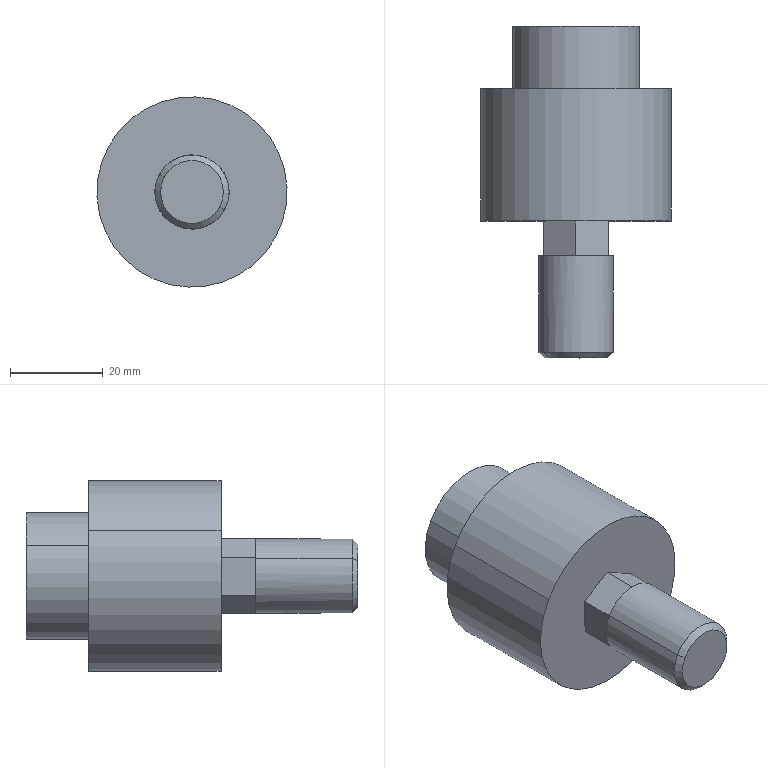Component | SolidWorks | FloatingJointSMCJA50-16-150-1 | 1 solid | 35 faces | box 41 x 71.5 x 41 mm | volume 48926 mm3 | plane 23 | cylinder 8 | cone 4 | commonest cylinder face diameters 41 x2 27.333 x2 16 x2 13.84 x2
STEP:
#1=CARTESIAN_POINT('',(0.08017,-1.417,7.279));
#2=VERTEX_POINT('',#1);
#3=CARTESIAN_POINT('',(1.495,-1.417,6.501));
#4=VERTEX_POINT('',#3);
#5=CARTESIAN_POINT('',(0.7874,-1.417,6.89));
#6=DIRECTION('',(-0.,1.,-0.));
#7=DIRECTION('',(-0.8763,0.,0.4818));
#8=AXIS2_PLACEMENT_3D('',#5,#6,#7);
#9=CIRCLE('',#8,0.8071);
#10=EDGE_CURVE('',#2,#4,#9,.T.);
#11=ORIENTED_EDGE('',*,*,#10,.T.);
#12=CARTESIAN_POINT('',(1.495,-0.2953,6.501));
#13=VERTEX_POINT('',#12);
#14=CARTESIAN_POINT('',(1.495,-0.8563,6.501));
#15=DIRECTION('',(-0.,1.,-0.));
#16=VECTOR('',#15,39.37);
#17=LINE('',#14,#16);
#18=EDGE_CURVE('',#4,#13,#17,.T.);
#19=ORIENTED_EDGE('',*,*,#18,.T.);
#20=CARTESIAN_POINT('',(0.08017,-0.2953,7.279));
#21=VERTEX_POINT('',#20);
#22=CARTESIAN_POINT('',(0.7874,-0.2953,6.89));
#23=DIRECTION('',(0.,-1.,0.));
#24=DIRECTION('',(-0.8763,0.,0.4818));
#25=AXIS2_PLACEMENT_3D('',#22,#23,#24);
#26=CIRCLE('',#25,0.8071);
#27=EDGE_CURVE('',#13,#21,#26,.T.);
#28=ORIENTED_EDGE('',*,*,#27,.T.);
#29=CARTESIAN_POINT('',(0.08017,-0.8563,7.279));
#30=DIRECTION('',(-0.,1.,-0.));
#31=VECTOR('',#30,39.37);
#32=LINE('',#29,#31);
#33=EDGE_CURVE('',#2,#21,#32,.T.);
#34=ORIENTED_EDGE('',*,*,#33,.F.);
#35=EDGE_LOOP('',(#11,#19,#28,#34));
#36=FACE_OUTER_BOUND('',#35,.T.);
#37=CARTESIAN_POINT('',(0.7874,-0.8563,6.89));
#38=DIRECTION('',(-0.,1.,-0.));
#39=DIRECTION('',(-0.8763,0.,0.4818));
#40=AXIS2_PLACEMENT_3D('',#37,#38,#39);
#41=CYLINDRICAL_SURFACE('',#40,0.8071);
#42=ADVANCED_FACE('',(#36),#41,.T.);
#43=CARTESIAN_POINT('',(1.259,-0.2953,6.631));
#44=VERTEX_POINT('',#43);
#45=CARTESIAN_POINT('',(0.3159,-0.2953,7.149));
#46=VERTEX_POINT('',#45);
#47=CARTESIAN_POINT('',(0.7874,-0.2953,6.89));
#48=DIRECTION('',(0.,-1.,0.));
#49=DIRECTION('',(-0.8763,0.,0.4818));
#50=AXIS2_PLACEMENT_3D('',#47,#48,#49);
#51=CIRCLE('',#50,0.5381);
#52=EDGE_CURVE('',#44,#46,#51,.T.);
#53=ORIENTED_EDGE('',*,*,#52,.F.);
#54=CARTESIAN_POINT('',(1.259,0.2362,6.631));
#55=VERTEX_POINT('',#54);
#56=CARTESIAN_POINT('',(1.259,-0.02953,6.631));
#57=DIRECTION('',(-0.,1.,-0.));
#58=VECTOR('',#57,39.37);
#59=LINE('',#56,#58);
#60=EDGE_CURVE('',#44,#55,#59,.T.);
#61=ORIENTED_EDGE('',*,*,#60,.T.);
#62=CARTESIAN_POINT('',(0.3159,0.2362,7.149));
#63=VERTEX_POINT('',#62);
#64=CARTESIAN_POINT('',(0.7874,0.2362,6.89));
#65=DIRECTION('',(0.,-1.,0.));
#66=DIRECTION('',(-0.8763,0.,0.4818));
#67=AXIS2_PLACEMENT_3D('',#64,#65,#66);
#68=CIRCLE('',#67,0.5381);
#69=EDGE_CURVE('',#55,#63,#68,.T.);
#70=ORIENTED_EDGE('',*,*,#69,.T.);
#71=CARTESIAN_POINT('',(0.3159,-0.02953,7.149));
#72=DIRECTION('',(-0.,1.,-0.));
#73=VECTOR('',#72,39.37);
#74=LINE('',#71,#73);
#75=EDGE_CURVE('',#46,#63,#74,.T.);
#76=ORIENTED_EDGE('',*,*,#75,.F.);
#77=EDGE_LOOP('',(#53,#61,#70,#76));
#78=FACE_OUTER_BOUND('',#77,.T.);
#79=CARTESIAN_POINT('',(0.7874,-0.02953,6.89));
#80=DIRECTION('',(-0.,1.,-0.));
#81=DIRECTION('',(-0.8763,0.,0.4818));
#82=AXIS2_PLACEMENT_3D('',#79,#80,#81);
#83=CYLINDRICAL_SURFACE('',#82,0.5381);
#84=ADVANCED_FACE('',(#78),#83,.T.);
#85=CARTESIAN_POINT('',(0.5114,-2.531,7.042));
#86=VERTEX_POINT('',#85);
#87=CARTESIAN_POINT('',(1.063,-2.531,6.738));
#88=VERTEX_POINT('',#87);
#89=CARTESIAN_POINT('',(0.7874,-2.531,6.89));
#90=DIRECTION('',(-0.,1.,-0.));
#91=DIRECTION('',(-0.8763,0.,0.4818));
#92=AXIS2_PLACEMENT_3D('',#89,#90,#91);
#93=CIRCLE('',#92,0.315);
#94=EDGE_CURVE('',#86,#88,#93,.T.);
#95=ORIENTED_EDGE('',*,*,#94,.T.);
#96=CARTESIAN_POINT('',(1.063,-1.713,6.738));
#97=VERTEX_POINT('',#96);
#98=CARTESIAN_POINT('',(1.063,-2.122,6.738));
#99=DIRECTION('',(-0.,1.,-0.));
#100=VECTOR('',#99,39.37);
#101=LINE('',#98,#100);
#102=EDGE_CURVE('',#88,#97,#101,.T.);
#103=ORIENTED_EDGE('',*,*,#102,.T.);
#104=CARTESIAN_POINT('',(1.066,-1.713,6.743));
#105=VERTEX_POINT('',#104);
#106=CARTESIAN_POINT('',(0.7874,-1.713,6.89));
#107=DIRECTION('',(-0.,1.,-0.));
#108=DIRECTION('',(-0.8763,0.,0.4818));
#109=AXIS2_PLACEMENT_3D('',#106,#107,#108);
#110=CIRCLE('',#109,0.315);
#111=EDGE_CURVE('',#105,#97,#110,.T.);
#112=ORIENTED_EDGE('',*,*,#111,.F.);
#113=CARTESIAN_POINT('',(1.06,-1.713,7.048));
#114=VERTEX_POINT('',#113);
#115=CARTESIAN_POINT('',(0.7874,-1.713,6.89));
#116=DIRECTION('',(-0.,1.,-0.));
#117=DIRECTION('',(-0.8763,0.,0.4818));
#118=AXIS2_PLACEMENT_3D('',#115,#116,#117);
#119=CIRCLE('',#118,0.315);
#120=EDGE_CURVE('',#114,#105,#119,.T.);
#121=ORIENTED_EDGE('',*,*,#120,.F.);
#122=CARTESIAN_POINT('',(1.054,-1.713,7.058));
#123=VERTEX_POINT('',#122);
#124=CARTESIAN_POINT('',(0.7874,-1.713,6.89));
#125=DIRECTION('',(-0.,1.,-0.));
#126=DIRECTION('',(-0.8763,0.,0.4818));
#127=AXIS2_PLACEMENT_3D('',#124,#125,#126);
#128=CIRCLE('',#127,0.315);
#129=EDGE_CURVE('',#123,#114,#128,.T.);
#130=ORIENTED_EDGE('',*,*,#129,.F.);
#131=CARTESIAN_POINT('',(0.7866,-1.713,7.205));
#132=VERTEX_POINT('',#131);
#133=CARTESIAN_POINT('',(0.7874,-1.713,6.89));
#134=DIRECTION('',(-0.,1.,-0.));
#135=DIRECTION('',(-0.8763,0.,0.4818));
#136=AXIS2_PLACEMENT_3D('',#133,#134,#135);
#137=CIRCLE('',#136,0.315);
#138=EDGE_CURVE('',#132,#123,#137,.T.);
#139=ORIENTED_EDGE('',*,*,#138,.F.);
#140=CARTESIAN_POINT('',(0.7751,-1.713,7.204));
#141=VERTEX_POINT('',#140);
#142=CARTESIAN_POINT('',(0.7874,-1.713,6.89));
#143=DIRECTION('',(-0.,1.,-0.));
#144=DIRECTION('',(-0.8763,0.,0.4818));
#145=AXIS2_PLACEMENT_3D('',#142,#143,#144);
#146=CIRCLE('',#145,0.315);
#147=EDGE_CURVE('',#141,#132,#146,.T.);
#148=ORIENTED_EDGE('',*,*,#147,.F.);
#149=CARTESIAN_POINT('',(0.5142,-1.713,7.047));
#150=VERTEX_POINT('',#149);
#151=CARTESIAN_POINT('',(0.7874,-1.713,6.89));
#152=DIRECTION('',(-0.,1.,-0.));
#153=DIRECTION('',(-0.8763,0.,0.4818));
#154=AXIS2_PLACEMENT_3D('',#151,#152,#153);
#155=CIRCLE('',#154,0.315);
#156=EDGE_CURVE('',#150,#141,#155,.T.);
#157=ORIENTED_EDGE('',*,*,#156,.F.);
#158=CARTESIAN_POINT('',(0.5114,-1.713,7.042));
#159=VERTEX_POINT('',#158);
#160=CARTESIAN_POINT('',(0.7874,-1.713,6.89));
#161=DIRECTION('',(-0.,1.,-0.));
#162=DIRECTION('',(-0.8763,0.,0.4818));
#163=AXIS2_PLACEMENT_3D('',#160,#161,#162);
#164=CIRCLE('',#163,0.315);
#165=EDGE_CURVE('',#159,#150,#164,.T.);
#166=ORIENTED_EDGE('',*,*,#165,.F.);
#167=CARTESIAN_POINT('',(0.5114,-2.122,7.042));
#168=DIRECTION('',(-0.,1.,-0.));
#169=VECTOR('',#168,39.37);
#170=LINE('',#167,#169);
#171=EDGE_CURVE('',#86,#159,#170,.T.);
#172=ORIENTED_EDGE('',*,*,#171,.F.);
#173=EDGE_LOOP('',(#95,#103,#112,#121,#130,#139,#148,#157,#166,#172));
#174=FACE_OUTER_BOUND('',#173,.T.);
#175=CARTESIAN_POINT('',(0.7874,-2.122,6.89));
#176=DIRECTION('',(-0.,1.,-0.));
#177=DIRECTION('',(-0.8763,0.,0.4818));
#178=AXIS2_PLACEMENT_3D('',#175,#176,#177);
#179=CYLINDRICAL_SURFACE('',#178,0.315);
#180=ADVANCED_FACE('',(#174),#179,.T.);
#181=CARTESIAN_POINT('',(1.026,0.1937,6.758));
#182=VERTEX_POINT('',#181);
#183=CARTESIAN_POINT('',(0.5487,0.1937,7.021));
#184=VERTEX_POINT('',#183);
#185=CARTESIAN_POINT('',(0.7874,0.1937,6.89));
#186=DIRECTION('',(-0.,1.,-0.));
#187=DIRECTION('',(0.4818,0.,0.8763));
#188=AXIS2_PLACEMENT_3D('',#185,#186,#187);
#189=CIRCLE('',#188,0.2724);
#190=EDGE_CURVE('',#182,#184,#189,.T.);
#191=ORIENTED_EDGE('',*,*,#190,.F.);
#192=CARTESIAN_POINT('',(1.063,0.2362,6.738));
#193=VERTEX_POINT('',#192);
#194=CARTESIAN_POINT('',(1.063,0.2362,6.738));
#195=DIRECTION('',(0.6196,0.7071,-0.3407));
#196=VECTOR('',#195,39.37);
#197=LINE('',#194,#196);
#198=EDGE_CURVE('',#182,#193,#197,.T.);
#199=ORIENTED_EDGE('',*,*,#198,.T.);
#200=CARTESIAN_POINT('',(0.5114,0.2362,7.042));
#201=VERTEX_POINT('',#200);
#202=CARTESIAN_POINT('',(0.7874,0.2362,6.89));
#203=DIRECTION('',(0.,-1.,0.));
#204=DIRECTION('',(-0.8763,0.,0.4818));
#205=AXIS2_PLACEMENT_3D('',#202,#203,#204);
#206=CIRCLE('',#205,0.315);
#207=EDGE_CURVE('',#201,#193,#206,.T.);
#208=ORIENTED_EDGE('',*,*,#207,.F.);
#209=CARTESIAN_POINT('',(0.5114,0.2362,7.042));
#210=DIRECTION('',(-0.6196,0.7071,0.3407));
#211=VECTOR('',#210,39.37);
#212=LINE('',#209,#211);
#213=EDGE_CURVE('',#184,#201,#212,.T.);
#214=ORIENTED_EDGE('',*,*,#213,.F.);
#215=EDGE_LOOP('',(#191,#199,#208,#214));
#216=FACE_OUTER_BOUND('',#215,.T.);
#217=CARTESIAN_POINT('',(0.7874,0.2362,6.89));
#218=DIRECTION('',(-0.,1.,-0.));
#219=DIRECTION('',(-0.8763,0.,0.4818));
#220=AXIS2_PLACEMENT_3D('',#217,#218,#219);
#221=CONICAL_SURFACE('',#220,0.315,0.7854);
#222=ADVANCED_FACE('',(#216),#221,.F.);
#223=CARTESIAN_POINT('',(0.5537,-2.579,7.018));
#224=VERTEX_POINT('',#223);
#225=CARTESIAN_POINT('',(1.021,-2.579,6.761));
#226=VERTEX_POINT('',#225);
#227=CARTESIAN_POINT('',(0.7874,-2.579,6.89));
#228=DIRECTION('',(-0.,1.,-0.));
#229=DIRECTION('',(-0.8763,0.,0.4818));
#230=AXIS2_PLACEMENT_3D('',#227,#228,#229);
#231=CIRCLE('',#230,0.2667);
#232=EDGE_CURVE('',#224,#226,#231,.T.);
#233=ORIENTED_EDGE('',*,*,#232,.T.);
#234=CARTESIAN_POINT('',(1.063,-2.531,6.738));
#235=DIRECTION('',(0.6196,0.7071,-0.3407));
#236=VECTOR('',#235,39.37);
#237=LINE('',#234,#236);
#238=EDGE_CURVE('',#226,#88,#237,.T.);
#239=ORIENTED_EDGE('',*,*,#238,.T.);
#240=ORIENTED_EDGE('',*,*,#94,.F.);
#241=CARTESIAN_POINT('',(0.5114,-2.531,7.042));
#242=DIRECTION('',(-0.6196,0.7071,0.3407));
#243=VECTOR('',#242,39.37);
#244=LINE('',#241,#243);
#245=EDGE_CURVE('',#224,#86,#244,.T.);
#246=ORIENTED_EDGE('',*,*,#245,.F.);
#247=EDGE_LOOP('',(#233,#239,#240,#246));
#248=FACE_OUTER_BOUND('',#247,.T.);
#249=CARTESIAN_POINT('',(0.7874,-2.531,6.89));
#250=DIRECTION('',(-0.,1.,-0.));
#251=DIRECTION('',(-0.8763,0.,0.4818));
#252=AXIS2_PLACEMENT_3D('',#249,#250,#251);
#253=CONICAL_SURFACE('',#252,0.315,0.7854);
#254=ADVANCED_FACE('',(#248),#253,.T.);
#255=CARTESIAN_POINT('',(1.026,-0.3543,6.758));
#256=VERTEX_POINT('',#255);
#257=CARTESIAN_POINT('',(0.5487,-0.3543,7.021));
#258=VERTEX_POINT('',#257);
#259=CARTESIAN_POINT('',(0.7874,-0.3543,6.89));
#260=DIRECTION('',(-0.,1.,-0.));
#261=DIRECTION('',(-0.8763,0.,0.4818));
#262=AXIS2_PLACEMENT_3D('',#259,#260,#261);
#263=CIRCLE('',#262,0.2724);
#264=EDGE_CURVE('',#256,#258,#263,.T.);
#265=ORIENTED_EDGE('',*,*,#264,.F.);
#266=CARTESIAN_POINT('',(1.026,-0.08031,6.758));
#267=DIRECTION('',(-0.,1.,-0.));
#268=VECTOR('',#267,39.37);
#269=LINE('',#266,#268);
#270=EDGE_CURVE('',#256,#182,#269,.T.);
#271=ORIENTED_EDGE('',*,*,#270,.T.);
#272=ORIENTED_EDGE('',*,*,#190,.T.);
#273=CARTESIAN_POINT('',(0.5487,-0.08031,7.021));
#274=DIRECTION('',(-0.,1.,-0.));
#275=VECTOR('',#274,39.37);
#276=LINE('',#273,#275);
#277=EDGE_CURVE('',#258,#184,#276,.T.);
#278=ORIENTED_EDGE('',*,*,#277,.F.);
#279=EDGE_LOOP('',(#265,#271,#272,#278));
#280=FACE_OUTER_BOUND('',#279,.T.);
#281=CARTESIAN_POINT('',(0.7874,-0.08031,6.89));
#282=DIRECTION('',(-0.,1.,-0.));
#283=DIRECTION('',(-0.8763,0.,0.4818));
#284=AXIS2_PLACEMENT_3D('',#281,#282,#283);
#285=CYLINDRICAL_SURFACE('',#284,0.2724);
#286=ADVANCED_FACE('',(#280),#285,.F.);
#287=ORIENTED_EDGE('',*,*,#18,.F.);
#288=CARTESIAN_POINT('',(0.7874,-1.417,6.89));
#289=DIRECTION('',(-0.,1.,-0.));
#290=DIRECTION('',(-0.8763,0.,0.4818));
#291=AXIS2_PLACEMENT_3D('',#288,#289,#290);
#292=CIRCLE('',#291,0.8071);
#293=EDGE_CURVE('',#4,#2,#292,.T.);
#294=ORIENTED_EDGE('',*,*,#293,.T.);
#295=ORIENTED_EDGE('',*,*,#33,.T.);
#296=CARTESIAN_POINT('',(0.7874,-0.2953,6.89));
#297=DIRECTION('',(0.,-1.,0.));
#298=DIRECTION('',(-0.8763,0.,0.4818));
#299=AXIS2_PLACEMENT_3D('',#296,#297,#298);
#300=CIRCLE('',#299,0.8071);
#301=EDGE_CURVE('',#21,#13,#300,.T.);
#302=ORIENTED_EDGE('',*,*,#301,.T.);
#303=EDGE_LOOP('',(#287,#294,#295,#302));
#304=FACE_OUTER_BOUND('',#303,.T.);
#305=CARTESIAN_POINT('',(0.7874,-0.8563,6.89));
#306=DIRECTION('',(-0.,1.,-0.));
#307=DIRECTION('',(-0.8763,0.,0.4818));
#308=AXIS2_PLACEMENT_3D('',#305,#306,#307);
#309=CYLINDRICAL_SURFACE('',#308,0.8071);
#310=ADVANCED_FACE('',(#304),#309,.T.);
#311=ORIENTED_EDGE('',*,*,#10,.F.);
#312=ORIENTED_EDGE('',*,*,#293,.F.);
#313=EDGE_LOOP('',(#311,#312));
#314=FACE_OUTER_BOUND('',#313,.T.);
#315=CARTESIAN_POINT('',(1.066,-1.417,6.736));
#316=VERTEX_POINT('',#315);
#317=CARTESIAN_POINT('',(0.794,-1.417,6.572));
#318=VERTEX_POINT('',#317);
#319=CARTESIAN_POINT('',(1.066,-1.417,6.736));
#320=DIRECTION('',(-0.8554,-0.,-0.518));
#321=VECTOR('',#320,39.37);
#322=LINE('',#319,#321);
#323=EDGE_CURVE('',#316,#318,#322,.T.);
#324=ORIENTED_EDGE('',*,*,#323,.T.);
#325=CARTESIAN_POINT('',(0.5152,-1.417,6.725));
#326=VERTEX_POINT('',#325);
#327=CARTESIAN_POINT('',(0.6546,-1.417,6.648));
#328=DIRECTION('',(-0.8763,0.,0.4818));
#329=VECTOR('',#328,39.37);
#330=LINE('',#327,#329);
#331=EDGE_CURVE('',#318,#326,#330,.T.);
#332=ORIENTED_EDGE('',*,*,#331,.T.);
#333=CARTESIAN_POINT('',(0.5086,-1.417,7.043));
#334=VERTEX_POINT('',#333);
#335=CARTESIAN_POINT('',(0.5152,-1.417,6.725));
#336=DIRECTION('',(-0.02087,0.,0.9998));
#337=VECTOR('',#336,39.37);
#338=LINE('',#335,#337);
#339=EDGE_CURVE('',#326,#334,#338,.T.);
#340=ORIENTED_EDGE('',*,*,#339,.T.);
#341=CARTESIAN_POINT('',(0.7808,-1.417,7.208));
#342=VERTEX_POINT('',#341);
#343=CARTESIAN_POINT('',(0.5086,-1.417,7.043));
#344=DIRECTION('',(0.8554,0.,0.518));
#345=VECTOR('',#344,39.37);
#346=LINE('',#343,#345);
#347=EDGE_CURVE('',#334,#342,#346,.T.);
#348=ORIENTED_EDGE('',*,*,#347,.T.);
#349=CARTESIAN_POINT('',(1.06,-1.417,7.055));
#350=VERTEX_POINT('',#349);
#351=CARTESIAN_POINT('',(0.9202,-1.417,7.131));
#352=DIRECTION('',(0.8763,-0.,-0.4818));
#353=VECTOR('',#352,39.37);
#354=LINE('',#351,#353);
#355=EDGE_CURVE('',#342,#350,#354,.T.);
#356=ORIENTED_EDGE('',*,*,#355,.T.);
#357=CARTESIAN_POINT('',(1.06,-1.417,7.055));
#358=DIRECTION('',(0.02087,-0.,-0.9998));
#359=VECTOR('',#358,39.37);
#360=LINE('',#357,#359);
#361=EDGE_CURVE('',#350,#316,#360,.T.);
#362=ORIENTED_EDGE('',*,*,#361,.T.);
#363=EDGE_LOOP('',(#324,#332,#340,#348,#356,#362));
#364=FACE_BOUND('',#363,.T.);
#365=CARTESIAN_POINT('',(0.9818,-1.417,7.243));
#366=DIRECTION('',(0.,-1.,0.));
#367=DIRECTION('',(0.8763,-0.,-0.4818));
#368=AXIS2_PLACEMENT_3D('',#365,#366,#367);
#369=PLANE('',#368);
#370=ADVANCED_FACE('',(#314,#364),#369,.T.);
#371=CARTESIAN_POINT('',(0.7874,-0.2953,6.89));
#372=DIRECTION('',(0.,-1.,0.));
#373=DIRECTION('',(-0.8763,0.,0.4818));
#374=AXIS2_PLACEMENT_3D('',#371,#372,#373);
#375=CIRCLE('',#374,0.5381);
#376=EDGE_CURVE('',#46,#44,#375,.T.);
#377=ORIENTED_EDGE('',*,*,#376,.T.);
#378=ORIENTED_EDGE('',*,*,#52,.T.);
#379=EDGE_LOOP('',(#377,#378));
#380=FACE_BOUND('',#379,.T.);
#381=ORIENTED_EDGE('',*,*,#301,.F.);
#382=ORIENTED_EDGE('',*,*,#27,.F.);
#383=EDGE_LOOP('',(#381,#382));
#384=FACE_OUTER_BOUND('',#383,.T.);
#385=CARTESIAN_POINT('',(1.111,-0.2953,7.479));
#386=DIRECTION('',(-0.,1.,-0.));
#387=DIRECTION('',(-0.8763,0.,0.4818));
#388=AXIS2_PLACEMENT_3D('',#385,#386,#387);
#389=PLANE('',#388);
#390=ADVANCED_FACE('',(#380,#384),#389,.T.);
#391=ORIENTED_EDGE('',*,*,#331,.F.);
#392=CARTESIAN_POINT('',(0.794,-1.713,6.572));
#393=VERTEX_POINT('',#392);
#394=CARTESIAN_POINT('',(0.794,-1.417,6.572));
#395=DIRECTION('',(0.,-1.,0.));
#396=VECTOR('',#395,39.37);
#397=LINE('',#394,#396);
#398=EDGE_CURVE('',#318,#393,#397,.T.);
#399=ORIENTED_EDGE('',*,*,#398,.T.);
#400=CARTESIAN_POINT('',(0.7882,-1.713,6.575));
#401=VERTEX_POINT('',#400);
#402=CARTESIAN_POINT('',(0.794,-1.713,6.572));
#403=DIRECTION('',(-0.8763,0.,0.4818));
#404=VECTOR('',#403,39.37);
#405=LINE('',#402,#404);
#406=EDGE_CURVE('',#393,#401,#405,.T.);
#407=ORIENTED_EDGE('',*,*,#406,.T.);
#408=CARTESIAN_POINT('',(0.521,-1.713,6.722));
#409=VERTEX_POINT('',#408);
#410=CARTESIAN_POINT('',(0.794,-1.713,6.572));
#411=DIRECTION('',(-0.8763,0.,0.4818));
#412=VECTOR('',#411,39.37);
#413=LINE('',#410,#412);
#414=EDGE_CURVE('',#401,#409,#413,.T.);
#415=ORIENTED_EDGE('',*,*,#414,.T.);
#416=CARTESIAN_POINT('',(0.5152,-1.713,6.725));
#417=VERTEX_POINT('',#416);
#418=CARTESIAN_POINT('',(0.794,-1.713,6.572));
#419=DIRECTION('',(-0.8763,0.,0.4818));
#420=VECTOR('',#419,39.37);
#421=LINE('',#418,#420);
#422=EDGE_CURVE('',#409,#417,#421,.T.);
#423=ORIENTED_EDGE('',*,*,#422,.T.);
#424=CARTESIAN_POINT('',(0.5152,-1.417,6.725));
#425=DIRECTION('',(-0.,1.,-0.));
#426=VECTOR('',#425,39.37);
#427=LINE('',#424,#426);
#428=EDGE_CURVE('',#417,#326,#427,.T.);
#429=ORIENTED_EDGE('',*,*,#428,.T.);
#430=EDGE_LOOP('',(#391,#399,#407,#415,#423,#429));
#431=FACE_OUTER_BOUND('',#430,.T.);
#432=CARTESIAN_POINT('',(0.794,-1.417,6.572));
#433=DIRECTION('',(-0.4818,-0.,-0.8763));
#434=DIRECTION('',(-0.,1.,-0.));
#435=AXIS2_PLACEMENT_3D('',#432,#433,#434);
#436=PLANE('',#435);
#437=ADVANCED_FACE('',(#431),#436,.T.);
#438=ORIENTED_EDGE('',*,*,#323,.F.);
#439=CARTESIAN_POINT('',(1.066,-1.713,6.736));
#440=VERTEX_POINT('',#439);
#441=CARTESIAN_POINT('',(1.066,-1.417,6.736));
#442=DIRECTION('',(0.,-1.,0.));
#443=VECTOR('',#442,39.37);
#444=LINE('',#441,#443);
#445=EDGE_CURVE('',#316,#440,#444,.T.);
#446=ORIENTED_EDGE('',*,*,#445,.T.);
#447=CARTESIAN_POINT('',(1.061,-1.713,6.733));
#448=VERTEX_POINT('',#447);
#449=CARTESIAN_POINT('',(1.066,-1.713,6.736));
#450=DIRECTION('',(-0.8554,-0.,-0.518));
#451=VECTOR('',#450,39.37);
#452=LINE('',#449,#451);
#453=EDGE_CURVE('',#440,#448,#452,.T.);
#454=ORIENTED_EDGE('',*,*,#453,.T.);
#455=CARTESIAN_POINT('',(0.7997,-1.713,6.575));
#456=VERTEX_POINT('',#455);
#457=CARTESIAN_POINT('',(1.066,-1.713,6.736));
#458=DIRECTION('',(-0.8554,-0.,-0.518));
#459=VECTOR('',#458,39.37);
#460=LINE('',#457,#459);
#461=EDGE_CURVE('',#448,#456,#460,.T.);
#462=ORIENTED_EDGE('',*,*,#461,.T.);
#463=CARTESIAN_POINT('',(1.066,-1.713,6.736));
#464=DIRECTION('',(-0.8554,-0.,-0.518));
#465=VECTOR('',#464,39.37);
#466=LINE('',#463,#465);
#467=EDGE_CURVE('',#456,#393,#466,.T.);
#468=ORIENTED_EDGE('',*,*,#467,.T.);
#469=ORIENTED_EDGE('',*,*,#398,.F.);
#470=EDGE_LOOP('',(#438,#446,#454,#462,#468,#469));
#471=FACE_OUTER_BOUND('',#470,.T.);
#472=CARTESIAN_POINT('',(1.066,-1.417,6.736));
#473=DIRECTION('',(0.518,-0.,-0.8554));
#474=DIRECTION('',(0.8554,0.,0.518));
#475=AXIS2_PLACEMENT_3D('',#472,#473,#474);
#476=PLANE('',#475);
#477=ADVANCED_FACE('',(#471),#476,.T.);
#478=ORIENTED_EDGE('',*,*,#361,.F.);
#479=CARTESIAN_POINT('',(1.06,-1.713,7.055));
#480=VERTEX_POINT('',#479);
#481=CARTESIAN_POINT('',(1.06,-1.417,7.055));
#482=DIRECTION('',(0.,-1.,0.));
#483=VECTOR('',#482,39.37);
#484=LINE('',#481,#483);
#485=EDGE_CURVE('',#350,#480,#484,.T.);
#486=ORIENTED_EDGE('',*,*,#485,.T.);
#487=CARTESIAN_POINT('',(1.06,-1.713,7.055));
#488=DIRECTION('',(0.02087,-0.,-0.9998));
#489=VECTOR('',#488,39.37);
#490=LINE('',#487,#489);
#491=EDGE_CURVE('',#480,#114,#490,.T.);
#492=ORIENTED_EDGE('',*,*,#491,.T.);
#493=CARTESIAN_POINT('',(1.06,-1.713,7.055));
#494=DIRECTION('',(0.02087,-0.,-0.9998));
#495=VECTOR('',#494,39.37);
#496=LINE('',#493,#495);
#497=EDGE_CURVE('',#114,#105,#496,.T.);
#498=ORIENTED_EDGE('',*,*,#497,.T.);
#499=CARTESIAN_POINT('',(1.06,-1.713,7.055));
#500=DIRECTION('',(0.02087,-0.,-0.9998));
#501=VECTOR('',#500,39.37);
#502=LINE('',#499,#501);
#503=EDGE_CURVE('',#105,#440,#502,.T.);
#504=ORIENTED_EDGE('',*,*,#503,.T.);
#505=ORIENTED_EDGE('',*,*,#445,.F.);
#506=EDGE_LOOP('',(#478,#486,#492,#498,#504,#505));
#507=FACE_OUTER_BOUND('',#506,.T.);
#508=CARTESIAN_POINT('',(1.06,-1.417,7.055));
#509=DIRECTION('',(0.9998,0.,0.02087));
#510=DIRECTION('',(-0.02087,0.,0.9998));
#511=AXIS2_PLACEMENT_3D('',#508,#509,#510);
#512=PLANE('',#511);
#513=ADVANCED_FACE('',(#507),#512,.T.);
#514=ORIENTED_EDGE('',*,*,#355,.F.);
#515=CARTESIAN_POINT('',(0.7808,-1.713,7.208));
#516=VERTEX_POINT('',#515);
#517=CARTESIAN_POINT('',(0.7808,-1.417,7.208));
#518=DIRECTION('',(0.,-1.,0.));
#519=VECTOR('',#518,39.37);
#520=LINE('',#517,#519);
#521=EDGE_CURVE('',#342,#516,#520,.T.);
#522=ORIENTED_EDGE('',*,*,#521,.T.);
#523=CARTESIAN_POINT('',(0.7808,-1.713,7.208));
#524=DIRECTION('',(0.8763,-0.,-0.4818));
#525=VECTOR('',#524,39.37);
#526=LINE('',#523,#525);
#527=EDGE_CURVE('',#516,#132,#526,.T.);
#528=ORIENTED_EDGE('',*,*,#527,.T.);
#529=CARTESIAN_POINT('',(0.7808,-1.713,7.208));
#530=DIRECTION('',(0.8763,-0.,-0.4818));
#531=VECTOR('',#530,39.37);
#532=LINE('',#529,#531);
#533=EDGE_CURVE('',#132,#123,#532,.T.);
#534=ORIENTED_EDGE('',*,*,#533,.T.);
#535=CARTESIAN_POINT('',(0.7808,-1.713,7.208));
#536=DIRECTION('',(0.8763,-0.,-0.4818));
#537=VECTOR('',#536,39.37);
#538=LINE('',#535,#537);
#539=EDGE_CURVE('',#123,#480,#538,.T.);
#540=ORIENTED_EDGE('',*,*,#539,.T.);
#541=ORIENTED_EDGE('',*,*,#485,.F.);
#542=EDGE_LOOP('',(#514,#522,#528,#534,#540,#541));
#543=FACE_OUTER_BOUND('',#542,.T.);
#544=CARTESIAN_POINT('',(0.7808,-1.417,7.208));
#545=DIRECTION('',(0.4818,0.,0.8763));
#546=DIRECTION('',(0.,-1.,0.));
#547=AXIS2_PLACEMENT_3D('',#544,#545,#546);
#548=PLANE('',#547);
#549=ADVANCED_FACE('',(#543),#548,.T.);
#550=ORIENTED_EDGE('',*,*,#347,.F.);
#551=CARTESIAN_POINT('',(0.5086,-1.713,7.043));
#552=VERTEX_POINT('',#551);
#553=CARTESIAN_POINT('',(0.5086,-1.417,7.043));
#554=DIRECTION('',(0.,-1.,0.));
#555=VECTOR('',#554,39.37);
#556=LINE('',#553,#555);
#557=EDGE_CURVE('',#334,#552,#556,.T.);
#558=ORIENTED_EDGE('',*,*,#557,.T.);
#559=CARTESIAN_POINT('',(0.5086,-1.713,7.043));
#560=DIRECTION('',(0.8554,0.,0.518));
#561=VECTOR('',#560,39.37);
#562=LINE('',#559,#561);
#563=EDGE_CURVE('',#552,#150,#562,.T.);
#564=ORIENTED_EDGE('',*,*,#563,.T.);
#565=CARTESIAN_POINT('',(0.5086,-1.713,7.043));
#566=DIRECTION('',(0.8554,0.,0.518));
#567=VECTOR('',#566,39.37);
#568=LINE('',#565,#567);
#569=EDGE_CURVE('',#150,#141,#568,.T.);
#570=ORIENTED_EDGE('',*,*,#569,.T.);
#571=CARTESIAN_POINT('',(0.5086,-1.713,7.043));
#572=DIRECTION('',(0.8554,0.,0.518));
#573=VECTOR('',#572,39.37);
#574=LINE('',#571,#573);
#575=EDGE_CURVE('',#141,#516,#574,.T.);
#576=ORIENTED_EDGE('',*,*,#575,.T.);
#577=ORIENTED_EDGE('',*,*,#521,.F.);
#578=EDGE_LOOP('',(#550,#558,#564,#570,#576,#577));
#579=FACE_OUTER_BOUND('',#578,.T.);
#580=CARTESIAN_POINT('',(0.5086,-1.417,7.043));
#581=DIRECTION('',(-0.518,0.,0.8554));
#582=DIRECTION('',(-0.8554,-0.,-0.518));
#583=AXIS2_PLACEMENT_3D('',#580,#581,#582);
#584=PLANE('',#583);
#585=ADVANCED_FACE('',(#579),#584,.T.);
#586=ORIENTED_EDGE('',*,*,#339,.F.);
#587=ORIENTED_EDGE('',*,*,#428,.F.);
#588=CARTESIAN_POINT('',(0.5151,-1.713,6.732));
#589=VERTEX_POINT('',#588);
#590=CARTESIAN_POINT('',(0.5152,-1.713,6.725));
#591=DIRECTION('',(-0.02087,0.,0.9998));
#592=VECTOR('',#591,39.37);
#593=LINE('',#590,#592);
#594=EDGE_CURVE('',#417,#589,#593,.T.);
#595=ORIENTED_EDGE('',*,*,#594,.T.);
#596=CARTESIAN_POINT('',(0.5087,-1.713,7.036));
#597=VERTEX_POINT('',#596);
#598=CARTESIAN_POINT('',(0.5152,-1.713,6.725));
#599=DIRECTION('',(-0.02087,0.,0.9998));
#600=VECTOR('',#599,39.37);
#601=LINE('',#598,#600);
#602=EDGE_CURVE('',#589,#597,#601,.T.);
#603=ORIENTED_EDGE('',*,*,#602,.T.);
#604=CARTESIAN_POINT('',(0.5152,-1.713,6.725));
#605=DIRECTION('',(-0.02087,0.,0.9998));
#606=VECTOR('',#605,39.37);
#607=LINE('',#604,#606);
#608=EDGE_CURVE('',#597,#552,#607,.T.);
#609=ORIENTED_EDGE('',*,*,#608,.T.);
#610=ORIENTED_EDGE('',*,*,#557,.F.);
#611=EDGE_LOOP('',(#586,#587,#595,#603,#609,#610));
#612=FACE_OUTER_BOUND('',#611,.T.);
#613=CARTESIAN_POINT('',(0.5152,-1.417,6.725));
#614=DIRECTION('',(-0.9998,-0.,-0.02087));
#615=DIRECTION('',(0.02087,-0.,-0.9998));
#616=AXIS2_PLACEMENT_3D('',#613,#614,#615);
#617=PLANE('',#616);
#618=ADVANCED_FACE('',(#612),#617,.T.);
#619=ORIENTED_EDGE('',*,*,#60,.F.);
#620=ORIENTED_EDGE('',*,*,#376,.F.);
#621=ORIENTED_EDGE('',*,*,#75,.T.);
#622=CARTESIAN_POINT('',(0.7874,0.2362,6.89));
#623=DIRECTION('',(0.,-1.,0.));
#624=DIRECTION('',(-0.8763,0.,0.4818));
#625=AXIS2_PLACEMENT_3D('',#622,#623,#624);
#626=CIRCLE('',#625,0.5381);
#627=EDGE_CURVE('',#63,#55,#626,.T.);
#628=ORIENTED_EDGE('',*,*,#627,.T.);
#629=EDGE_LOOP('',(#619,#620,#621,#628));
#630=FACE_OUTER_BOUND('',#629,.T.);
#631=CARTESIAN_POINT('',(0.7874,-0.02953,6.89));
#632=DIRECTION('',(-0.,1.,-0.));
#633=DIRECTION('',(-0.8763,0.,0.4818));
#634=AXIS2_PLACEMENT_3D('',#631,#632,#633);
#635=CYLINDRICAL_SURFACE('',#634,0.5381);
#636=ADVANCED_FACE('',(#630),#635,.T.);
#637=ORIENTED_EDGE('',*,*,#594,.F.);
#638=ORIENTED_EDGE('',*,*,#422,.F.);
#639=CARTESIAN_POINT('',(0.7874,-1.713,6.89));
#640=DIRECTION('',(0.,-1.,0.));
#641=DIRECTION('',(-0.8763,0.,0.4818));
#642=AXIS2_PLACEMENT_3D('',#639,#640,#641);
#643=CIRCLE('',#642,0.315);
#644=EDGE_CURVE('',#589,#409,#643,.T.);
#645=ORIENTED_EDGE('',*,*,#644,.F.);
#646=EDGE_LOOP('',(#637,#638,#645));
#647=FACE_OUTER_BOUND('',#646,.T.);
#648=CARTESIAN_POINT('',(0.7874,-1.713,6.89));
#649=DIRECTION('',(0.,-1.,0.));
#650=DIRECTION('',(0.8763,-0.,-0.4818));
#651=AXIS2_PLACEMENT_3D('',#648,#649,#650);
#652=PLANE('',#651);
#653=ADVANCED_FACE('',(#647),#652,.T.);
#654=ORIENTED_EDGE('',*,*,#414,.F.);
#655=CARTESIAN_POINT('',(0.7874,-1.713,6.89));
#656=DIRECTION('',(-0.,1.,-0.));
#657=DIRECTION('',(-0.8763,0.,0.4818));
#658=AXIS2_PLACEMENT_3D('',#655,#656,#657);
#659=CIRCLE('',#658,0.315);
#660=EDGE_CURVE('',#401,#409,#659,.T.);
#661=ORIENTED_EDGE('',*,*,#660,.T.);
#662=EDGE_LOOP('',(#654,#661));
#663=FACE_OUTER_BOUND('',#662,.T.);
#664=CARTESIAN_POINT('',(0.8633,-1.713,7.028));
#665=DIRECTION('',(-0.,1.,-0.));
#666=DIRECTION('',(-0.8763,0.,0.4818));
#667=AXIS2_PLACEMENT_3D('',#664,#665,#666);
#668=PLANE('',#667);
#669=ADVANCED_FACE('',(#663),#668,.T.);
#670=ORIENTED_EDGE('',*,*,#406,.F.);
#671=ORIENTED_EDGE('',*,*,#467,.F.);
#672=CARTESIAN_POINT('',(0.7874,-1.713,6.89));
#673=DIRECTION('',(-0.,1.,-0.));
#674=DIRECTION('',(-0.8763,0.,0.4818));
#675=AXIS2_PLACEMENT_3D('',#672,#673,#674);
#676=CIRCLE('',#675,0.315);
#677=EDGE_CURVE('',#456,#401,#676,.T.);
#678=ORIENTED_EDGE('',*,*,#677,.T.);
#679=EDGE_LOOP('',(#670,#671,#678));
#680=FACE_OUTER_BOUND('',#679,.T.);
#681=CARTESIAN_POINT('',(0.7874,-1.713,6.89));
#682=DIRECTION('',(0.,-1.,0.));
#683=DIRECTION('',(0.8763,-0.,-0.4818));
#684=AXIS2_PLACEMENT_3D('',#681,#682,#683);
#685=PLANE('',#684);
#686=ADVANCED_FACE('',(#680),#685,.T.);
#687=ORIENTED_EDGE('',*,*,#461,.F.);
#688=CARTESIAN_POINT('',(0.7874,-1.713,6.89));
#689=DIRECTION('',(-0.,1.,-0.));
#690=DIRECTION('',(-0.8763,0.,0.4818));
#691=AXIS2_PLACEMENT_3D('',#688,#689,#690);
#692=CIRCLE('',#691,0.315);
#693=EDGE_CURVE('',#448,#456,#692,.T.);
#694=ORIENTED_EDGE('',*,*,#693,.T.);
#695=EDGE_LOOP('',(#687,#694));
#696=FACE_OUTER_BOUND('',#695,.T.);
#697=CARTESIAN_POINT('',(0.8633,-1.713,7.028));
#698=DIRECTION('',(-0.,1.,-0.));
#699=DIRECTION('',(-0.8763,0.,0.4818));
#700=AXIS2_PLACEMENT_3D('',#697,#698,#699);
#701=PLANE('',#700);
#702=ADVANCED_FACE('',(#696),#701,.T.);
#703=ORIENTED_EDGE('',*,*,#453,.F.);
#704=ORIENTED_EDGE('',*,*,#503,.F.);
#705=ORIENTED_EDGE('',*,*,#111,.T.);
#706=CARTESIAN_POINT('',(0.7874,-1.713,6.89));
#707=DIRECTION('',(-0.,1.,-0.));
#708=DIRECTION('',(-0.8763,0.,0.4818));
#709=AXIS2_PLACEMENT_3D('',#706,#707,#708);
#710=CIRCLE('',#709,0.315);
#711=EDGE_CURVE('',#97,#448,#710,.T.);
#712=ORIENTED_EDGE('',*,*,#711,.T.);
#713=EDGE_LOOP('',(#703,#704,#705,#712));
#714=FACE_OUTER_BOUND('',#713,.T.);
#715=CARTESIAN_POINT('',(0.7874,-1.713,6.89));
#716=DIRECTION('',(0.,-1.,0.));
#717=DIRECTION('',(0.8763,-0.,-0.4818));
#718=AXIS2_PLACEMENT_3D('',#715,#716,#717);
#719=PLANE('',#718);
#720=ADVANCED_FACE('',(#714),#719,.T.);
#721=ORIENTED_EDGE('',*,*,#497,.F.);
#722=ORIENTED_EDGE('',*,*,#120,.T.);
#723=EDGE_LOOP('',(#721,#722));
#724=FACE_OUTER_BOUND('',#723,.T.);
#725=CARTESIAN_POINT('',(0.8633,-1.713,7.028));
#726=DIRECTION('',(-0.,1.,-0.));
#727=DIRECTION('',(-0.8763,0.,0.4818));
#728=AXIS2_PLACEMENT_3D('',#725,#726,#727);
#729=PLANE('',#728);
#730=ADVANCED_FACE('',(#724),#729,.T.);
#731=ORIENTED_EDGE('',*,*,#491,.F.);
#732=ORIENTED_EDGE('',*,*,#539,.F.);
#733=ORIENTED_EDGE('',*,*,#129,.T.);
#734=EDGE_LOOP('',(#731,#732,#733));
#735=FACE_OUTER_BOUND('',#734,.T.);
#736=CARTESIAN_POINT('',(0.7874,-1.713,6.89));
#737=DIRECTION('',(0.,-1.,0.));
#738=DIRECTION('',(0.8763,-0.,-0.4818));
#739=AXIS2_PLACEMENT_3D('',#736,#737,#738);
#740=PLANE('',#739);
#741=ADVANCED_FACE('',(#735),#740,.T.);
#742=ORIENTED_EDGE('',*,*,#533,.F.);
#743=ORIENTED_EDGE('',*,*,#138,.T.);
#744=EDGE_LOOP('',(#742,#743));
#745=FACE_OUTER_BOUND('',#744,.T.);
#746=CARTESIAN_POINT('',(0.8633,-1.713,7.028));
#747=DIRECTION('',(-0.,1.,-0.));
#748=DIRECTION('',(-0.8763,0.,0.4818));
#749=AXIS2_PLACEMENT_3D('',#746,#747,#748);
#750=PLANE('',#749);
#751=ADVANCED_FACE('',(#745),#750,.T.);
#752=ORIENTED_EDGE('',*,*,#527,.F.);
#753=ORIENTED_EDGE('',*,*,#575,.F.);
#754=ORIENTED_EDGE('',*,*,#147,.T.);
#755=EDGE_LOOP('',(#752,#753,#754));
#756=FACE_OUTER_BOUND('',#755,.T.);
#757=CARTESIAN_POINT('',(0.7874,-1.713,6.89));
#758=DIRECTION('',(0.,-1.,0.));
#759=DIRECTION('',(0.8763,-0.,-0.4818));
#760=AXIS2_PLACEMENT_3D('',#757,#758,#759);
#761=PLANE('',#760);
#762=ADVANCED_FACE('',(#756),#761,.T.);
#763=ORIENTED_EDGE('',*,*,#569,.F.);
#764=ORIENTED_EDGE('',*,*,#156,.T.);
#765=EDGE_LOOP('',(#763,#764));
#766=FACE_OUTER_BOUND('',#765,.T.);
#767=CARTESIAN_POINT('',(0.8633,-1.713,7.028));
#768=DIRECTION('',(-0.,1.,-0.));
#769=DIRECTION('',(-0.8763,0.,0.4818));
#770=AXIS2_PLACEMENT_3D('',#767,#768,#769);
#771=PLANE('',#770);
#772=ADVANCED_FACE('',(#766),#771,.T.);
#773=ORIENTED_EDGE('',*,*,#563,.F.);
#774=ORIENTED_EDGE('',*,*,#608,.F.);
#775=CARTESIAN_POINT('',(0.7874,-1.713,6.89));
#776=DIRECTION('',(-0.,1.,-0.));
#777=DIRECTION('',(-0.8763,0.,0.4818));
#778=AXIS2_PLACEMENT_3D('',#775,#776,#777);
#779=CIRCLE('',#778,0.315);
#780=EDGE_CURVE('',#597,#159,#779,.T.);
#781=ORIENTED_EDGE('',*,*,#780,.T.);
#782=ORIENTED_EDGE('',*,*,#165,.T.);
#783=EDGE_LOOP('',(#773,#774,#781,#782));
#784=FACE_OUTER_BOUND('',#783,.T.);
#785=CARTESIAN_POINT('',(0.7874,-1.713,6.89));
#786=DIRECTION('',(0.,-1.,0.));
#787=DIRECTION('',(0.8763,-0.,-0.4818));
#788=AXIS2_PLACEMENT_3D('',#785,#786,#787);
#789=PLANE('',#788);
#790=ADVANCED_FACE('',(#784),#789,.T.);
#791=ORIENTED_EDGE('',*,*,#602,.F.);
#792=CARTESIAN_POINT('',(0.7874,-1.713,6.89));
#793=DIRECTION('',(-0.,1.,-0.));
#794=DIRECTION('',(-0.8763,0.,0.4818));
#795=AXIS2_PLACEMENT_3D('',#792,#793,#794);
#796=CIRCLE('',#795,0.315);
#797=EDGE_CURVE('',#589,#597,#796,.T.);
#798=ORIENTED_EDGE('',*,*,#797,.T.);
#799=EDGE_LOOP('',(#791,#798));
#800=FACE_OUTER_BOUND('',#799,.T.);
#801=CARTESIAN_POINT('',(0.8633,-1.713,7.028));
#802=DIRECTION('',(-0.,1.,-0.));
#803=DIRECTION('',(-0.8763,0.,0.4818));
#804=AXIS2_PLACEMENT_3D('',#801,#802,#803);
#805=PLANE('',#804);
#806=ADVANCED_FACE('',(#800),#805,.T.);
#807=ORIENTED_EDGE('',*,*,#207,.T.);
#808=CARTESIAN_POINT('',(0.7874,0.2362,6.89));
#809=DIRECTION('',(0.,-1.,0.));
#810=DIRECTION('',(-0.8763,0.,0.4818));
#811=AXIS2_PLACEMENT_3D('',#808,#809,#810);
#812=CIRCLE('',#811,0.315);
#813=EDGE_CURVE('',#193,#201,#812,.T.);
#814=ORIENTED_EDGE('',*,*,#813,.T.);
#815=EDGE_LOOP('',(#807,#814));
#816=FACE_BOUND('',#815,.T.);
#817=ORIENTED_EDGE('',*,*,#627,.F.);
#818=ORIENTED_EDGE('',*,*,#69,.F.);
#819=EDGE_LOOP('',(#817,#818));
#820=FACE_OUTER_BOUND('',#819,.T.);
#821=CARTESIAN_POINT('',(0.9929,0.2362,7.264));
#822=DIRECTION('',(-0.,1.,-0.));
#823=DIRECTION('',(-0.8763,0.,0.4818));
#824=AXIS2_PLACEMENT_3D('',#821,#822,#823);
#825=PLANE('',#824);
#826=ADVANCED_FACE('',(#816,#820),#825,.T.);
#827=ORIENTED_EDGE('',*,*,#102,.F.);
#828=CARTESIAN_POINT('',(0.7874,-2.531,6.89));
#829=DIRECTION('',(-0.,1.,-0.));
#830=DIRECTION('',(-0.8763,0.,0.4818));
#831=AXIS2_PLACEMENT_3D('',#828,#829,#830);
#832=CIRCLE('',#831,0.315);
#833=EDGE_CURVE('',#88,#86,#832,.T.);
#834=ORIENTED_EDGE('',*,*,#833,.T.);
#835=ORIENTED_EDGE('',*,*,#171,.T.);
#836=ORIENTED_EDGE('',*,*,#780,.F.);
#837=ORIENTED_EDGE('',*,*,#797,.F.);
#838=ORIENTED_EDGE('',*,*,#644,.T.);
#839=ORIENTED_EDGE('',*,*,#660,.F.);
#840=ORIENTED_EDGE('',*,*,#677,.F.);
#841=ORIENTED_EDGE('',*,*,#693,.F.);
#842=ORIENTED_EDGE('',*,*,#711,.F.);
#843=EDGE_LOOP('',(#827,#834,#835,#836,#837,#838,#839,#840,#841,#842));
#844=FACE_OUTER_BOUND('',#843,.T.);
#845=CARTESIAN_POINT('',(0.7874,-2.122,6.89));
#846=DIRECTION('',(-0.,1.,-0.));
#847=DIRECTION('',(-0.8763,0.,0.4818));
#848=AXIS2_PLACEMENT_3D('',#845,#846,#847);
#849=CYLINDRICAL_SURFACE('',#848,0.315);
#850=ADVANCED_FACE('',(#844),#849,.T.);
#851=ORIENTED_EDGE('',*,*,#198,.F.);
#852=CARTESIAN_POINT('',(0.7874,0.1937,6.89));
#853=DIRECTION('',(-0.,1.,-0.));
#854=DIRECTION('',(0.4818,0.,0.8763));
#855=AXIS2_PLACEMENT_3D('',#852,#853,#854);
#856=CIRCLE('',#855,0.2724);
#857=EDGE_CURVE('',#184,#182,#856,.T.);
#858=ORIENTED_EDGE('',*,*,#857,.F.);
#859=ORIENTED_EDGE('',*,*,#213,.T.);
#860=ORIENTED_EDGE('',*,*,#813,.F.);
#861=EDGE_LOOP('',(#851,#858,#859,#860));
#862=FACE_OUTER_BOUND('',#861,.T.);
#863=CARTESIAN_POINT('',(0.7874,0.2362,6.89));
#864=DIRECTION('',(-0.,1.,-0.));
#865=DIRECTION('',(-0.8763,0.,0.4818));
#866=AXIS2_PLACEMENT_3D('',#863,#864,#865);
#867=CONICAL_SURFACE('',#866,0.315,0.7854);
#868=ADVANCED_FACE('',(#862),#867,.F.);
#869=ORIENTED_EDGE('',*,*,#238,.F.);
#870=CARTESIAN_POINT('',(0.7874,-2.579,6.89));
#871=DIRECTION('',(-0.,1.,-0.));
#872=DIRECTION('',(-0.8763,0.,0.4818));
#873=AXIS2_PLACEMENT_3D('',#870,#871,#872);
#874=CIRCLE('',#873,0.2667);
#875=EDGE_CURVE('',#226,#224,#874,.T.);
#876=ORIENTED_EDGE('',*,*,#875,.T.);
#877=ORIENTED_EDGE('',*,*,#245,.T.);
#878=ORIENTED_EDGE('',*,*,#833,.F.);
#879=EDGE_LOOP('',(#869,#876,#877,#878));
#880=FACE_OUTER_BOUND('',#879,.T.);
#881=CARTESIAN_POINT('',(0.7874,-2.531,6.89));
#882=DIRECTION('',(-0.,1.,-0.));
#883=DIRECTION('',(-0.8763,0.,0.4818));
#884=AXIS2_PLACEMENT_3D('',#881,#882,#883);
#885=CONICAL_SURFACE('',#884,0.315,0.7854);
#886=ADVANCED_FACE('',(#880),#885,.T.);
#887=ORIENTED_EDGE('',*,*,#270,.F.);
#888=CARTESIAN_POINT('',(0.7874,-0.3543,6.89));
#889=DIRECTION('',(-0.,1.,-0.));
#890=DIRECTION('',(-0.8763,0.,0.4818));
#891=AXIS2_PLACEMENT_3D('',#888,#889,#890);
#892=CIRCLE('',#891,0.2724);
#893=EDGE_CURVE('',#258,#256,#892,.T.);
#894=ORIENTED_EDGE('',*,*,#893,.F.);
#895=ORIENTED_EDGE('',*,*,#277,.T.);
#896=ORIENTED_EDGE('',*,*,#857,.T.);
#897=EDGE_LOOP('',(#887,#894,#895,#896));
#898=FACE_OUTER_BOUND('',#897,.T.);
#899=CARTESIAN_POINT('',(0.7874,-0.08031,6.89));
#900=DIRECTION('',(-0.,1.,-0.));
#901=DIRECTION('',(-0.8763,0.,0.4818));
#902=AXIS2_PLACEMENT_3D('',#899,#900,#901);
#903=CYLINDRICAL_SURFACE('',#902,0.2724);
#904=ADVANCED_FACE('',(#898),#903,.F.);
#905=ORIENTED_EDGE('',*,*,#232,.F.);
#906=ORIENTED_EDGE('',*,*,#875,.F.);
#907=EDGE_LOOP('',(#905,#906));
#908=FACE_OUTER_BOUND('',#907,.T.);
#909=CARTESIAN_POINT('',(0.8517,-2.579,7.007));
#910=DIRECTION('',(0.,-1.,0.));
#911=DIRECTION('',(0.8763,-0.,-0.4818));
#912=AXIS2_PLACEMENT_3D('',#909,#910,#911);
#913=PLANE('',#912);
#914=ADVANCED_FACE('',(#908),#913,.T.);
#915=ORIENTED_EDGE('',*,*,#893,.T.);
#916=ORIENTED_EDGE('',*,*,#264,.T.);
#917=EDGE_LOOP('',(#915,#916));
#918=FACE_OUTER_BOUND('',#917,.T.);
#919=CARTESIAN_POINT('',(0.853,-0.3543,7.009));
#920=DIRECTION('',(-0.,1.,-0.));
#921=DIRECTION('',(-0.8763,0.,0.4818));
#922=AXIS2_PLACEMENT_3D('',#919,#920,#921);
#923=PLANE('',#922);
#924=ADVANCED_FACE('',(#918),#923,.T.);
#925=CLOSED_SHELL('',(#42,#84,#180,#222,#254,#286,#310,#370,#390,#437,#477,#513,#549,#585,#618,#636,#653,#669,#686,#702,#720,#730,#741,#751,#762,#772,#790,#806,#826,#850,#868,#886,#904,#914,#924));
#926=MANIFOLD_SOLID_BREP('',#925);
#927=CARTESIAN_POINT('',(0.,0.,0.));
#928=DIRECTION('',(0.,0.,1.));
#929=DIRECTION('',(1.,0.,0.));
#930=AXIS2_PLACEMENT_3D('',#927,#928,#929);
#931=(LENGTH_UNIT()NAMED_UNIT(*)SI_UNIT($,.METRE.));
#932=LENGTH_MEASURE_WITH_UNIT(LENGTH_MEASURE(0.0254),#931);
#933=DIMENSIONAL_EXPONENTS(1.,0.,0.,0.,0.,0.,0.);
#934=(CONVERSION_BASED_UNIT('',#932)LENGTH_UNIT()NAMED_UNIT(#933));
#935=UNCERTAINTY_MEASURE_WITH_UNIT(LENGTH_MEASURE(0.00001),#934,'','');
#936=(NAMED_UNIT(*)PLANE_ANGLE_UNIT()SI_UNIT($,.RADIAN.));
#937=(NAMED_UNIT(*)SI_UNIT($,.STERADIAN.)SOLID_ANGLE_UNIT());
#938=(GEOMETRIC_REPRESENTATION_CONTEXT(3)GLOBAL_UNCERTAINTY_ASSIGNED_CONTEXT((#935))GLOBAL_UNIT_ASSIGNED_CONTEXT((#934,#936,#937))REPRESENTATION_CONTEXT('',''));
#939=ADVANCED_BREP_SHAPE_REPRESENTATION('',(#926,#930),#938);
#940=COLOUR_RGB('',0.7922,0.8196,0.9333);
#941=FILL_AREA_STYLE_COLOUR('',#940);
#942=FILL_AREA_STYLE('',(#941));
#943=SURFACE_STYLE_FILL_AREA(#942);
#944=SURFACE_SIDE_STYLE('',(#943));
#945=SURFACE_STYLE_USAGE(.BOTH.,#944);
#946=PRESENTATION_STYLE_ASSIGNMENT((#945));
#947=STYLED_ITEM('',(#946),#926);
#948=PRESENTATION_LAYER_ASSIGNMENT('','',(#947));
#949=(LENGTH_UNIT()NAMED_UNIT(*)SI_UNIT($,.METRE.));
#950=LENGTH_MEASURE_WITH_UNIT(LENGTH_MEASURE(0.0254),#949);
#951=DIMENSIONAL_EXPONENTS(1.,0.,0.,0.,0.,0.,0.);
#952=(CONVERSION_BASED_UNIT('',#950)LENGTH_UNIT()NAMED_UNIT(#951));
#953=UNCERTAINTY_MEASURE_WITH_UNIT(LENGTH_MEASURE(0.00001),#952,'','');
#954=(NAMED_UNIT(*)PLANE_ANGLE_UNIT()SI_UNIT($,.RADIAN.));
#955=(NAMED_UNIT(*)SI_UNIT($,.STERADIAN.)SOLID_ANGLE_UNIT());
#956=(GEOMETRIC_REPRESENTATION_CONTEXT(3)GLOBAL_UNCERTAINTY_ASSIGNED_CONTEXT((#953))GLOBAL_UNIT_ASSIGNED_CONTEXT((#952,#954,#955))REPRESENTATION_CONTEXT('',''));
#957=MECHANICAL_DESIGN_GEOMETRIC_PRESENTATION_REPRESENTATION('',(#947),#956);